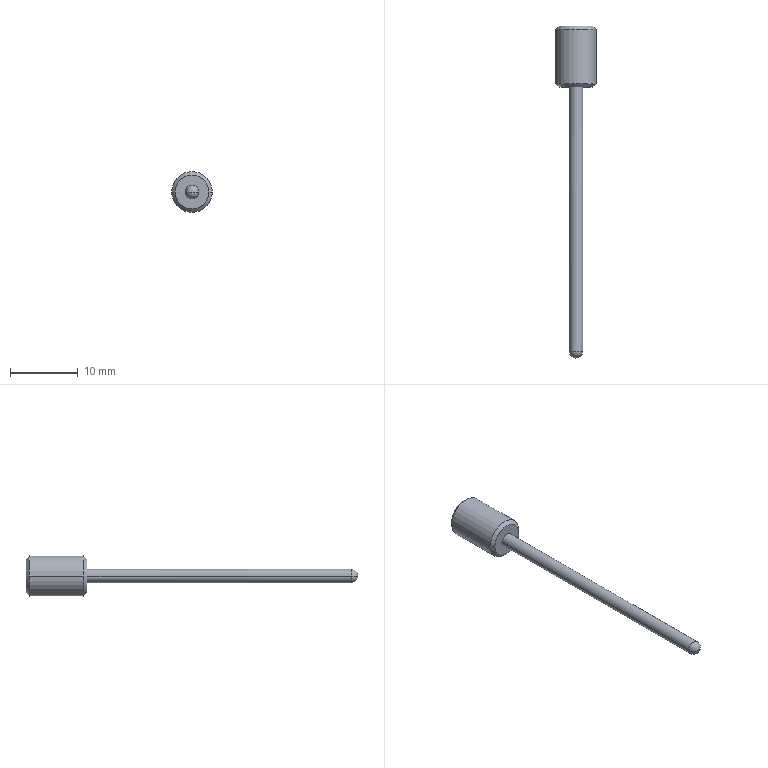Component | SolidWorks | TeaSortingRod-1 | 1 solid | 16 faces | box 6 x 49 x 6 mm | volume 309 mm3 | cone 6 | cylinder 6 | sphere 2 | plane 2 | commonest cylinder face diameters 3.3 x2 2 x2 6 x2
build123d program:
from build123d import *

# Parameters (mm, degrees)
SKETCH1_R             = 3
BOSS_EXTRUDE1_DEPTH   = 9
SKETCH2_R             = 1
BOSS_EXTRUDE2_DEPTH   = 40
M4_TAPPED_HOLE1_D     = 3.3
M4_TAPPED_HOLE1_DEPTH = 7.1
M4_TAPPED_HOLE1_TIP   = 1.65
FILLET1_R             = 1
CHAMFER1_SIZE         = 0.5


with BuildPart() as part:
    # Sketch1 → Boss-Extrude1 (new body)
    with BuildSketch(Plane.XY):
        Circle(SKETCH1_R)
    extrude(amount=BOSS_EXTRUDE1_DEPTH)

    # Sketch2 → Boss-Extrude2 (add)
    with BuildSketch(Plane.XY.offset(9)):
        Circle(SKETCH2_R)
    extrude(amount=BOSS_EXTRUDE2_DEPTH)

    # M4 Tapped Hole1
    with Locations(Plane(origin=(0, 0, 0), x_dir=(-1, 0, 0), z_dir=(0, 0, -1))):
        with Locations((0, 0)):
            Hole(M4_TAPPED_HOLE1_D / 2, depth=M4_TAPPED_HOLE1_DEPTH)
            with Locations((0, 0, -(M4_TAPPED_HOLE1_DEPTH + M4_TAPPED_HOLE1_TIP / 2))):  # 90° drill point
                Cone(0, M4_TAPPED_HOLE1_D / 2, M4_TAPPED_HOLE1_TIP, mode=Mode.SUBTRACT)

    # Fillet1
    fillet1_edges = [part.edges().sort_by_distance(p)[0] for p in [
        (-1, 0, 49),
    ]]
    fillet(fillet1_edges, radius=FILLET1_R)

    # Chamfer1
    chamfer1_edges = [part.edges().sort_by_distance(p)[0] for p in [
        (-3, 0, 0),
        (-3, 0, 9),
    ]]
    chamfer(chamfer1_edges, length=CHAMFER1_SIZE)


solid = part.part

# Placed as in the assembly
solid = solid.moved(Location((64.354, -142.761, 166.933), (90, 0, 0)))
STEP:
#1=COLOUR_RGB('',0.7922,0.8196,0.9333);
#2=FILL_AREA_STYLE_COLOUR('',#1);
#3=FILL_AREA_STYLE('',(#2));
#4=SURFACE_STYLE_FILL_AREA(#3);
#5=SURFACE_SIDE_STYLE('',(#4));
#6=SURFACE_STYLE_USAGE(.BOTH.,#5);
#7=PRESENTATION_STYLE_ASSIGNMENT((#6));
#8=CARTESIAN_POINT('',(2.632,-5.975,6.572));
#9=VERTEX_POINT('',#8);
#10=CARTESIAN_POINT('',(2.435,-5.975,6.572));
#11=VERTEX_POINT('',#10);
#12=CARTESIAN_POINT('',(2.534,-5.975,6.572));
#13=DIRECTION('',(-0.,-1.,-0.));
#14=DIRECTION('',(1.,0.,0.));
#15=AXIS2_PLACEMENT_3D('',#12,#13,#14);
#16=CIRCLE('',#15,0.09843);
#17=EDGE_CURVE('',#9,#11,#16,.T.);
#18=ORIENTED_EDGE('',*,*,#17,.F.);
#19=CARTESIAN_POINT('',(2.652,-5.955,6.572));
#20=VERTEX_POINT('',#19);
#21=CARTESIAN_POINT('',(2.632,-5.975,6.572));
#22=DIRECTION('',(0.7071,0.7071,0.));
#23=VECTOR('',#22,39.37);
#24=LINE('',#21,#23);
#25=EDGE_CURVE('',#9,#20,#24,.T.);
#26=ORIENTED_EDGE('',*,*,#25,.T.);
#27=CARTESIAN_POINT('',(2.416,-5.955,6.572));
#28=VERTEX_POINT('',#27);
#29=CARTESIAN_POINT('',(2.534,-5.955,6.572));
#30=DIRECTION('',(0.,1.,0.));
#31=DIRECTION('',(1.,0.,0.));
#32=AXIS2_PLACEMENT_3D('',#29,#30,#31);
#33=CIRCLE('',#32,0.1181);
#34=EDGE_CURVE('',#28,#20,#33,.T.);
#35=ORIENTED_EDGE('',*,*,#34,.F.);
#36=CARTESIAN_POINT('',(2.435,-5.975,6.572));
#37=DIRECTION('',(-0.7071,0.7071,-0.));
#38=VECTOR('',#37,39.37);
#39=LINE('',#36,#38);
#40=EDGE_CURVE('',#11,#28,#39,.T.);
#41=ORIENTED_EDGE('',*,*,#40,.F.);
#42=EDGE_LOOP('',(#18,#26,#35,#41));
#43=FACE_OUTER_BOUND('',#42,.T.);
#44=CARTESIAN_POINT('',(2.534,-5.975,6.572));
#45=DIRECTION('',(0.,1.,0.));
#46=DIRECTION('',(-1.,0.,0.));
#47=AXIS2_PLACEMENT_3D('',#44,#45,#46);
#48=CONICAL_SURFACE('',#47,0.09843,0.7854);
#49=ADVANCED_FACE('',(#43),#48,.T.);
#50=CARTESIAN_POINT('',(2.435,-5.621,6.572));
#51=VERTEX_POINT('',#50);
#52=CARTESIAN_POINT('',(2.632,-5.621,6.572));
#53=VERTEX_POINT('',#52);
#54=CARTESIAN_POINT('',(2.534,-5.621,6.572));
#55=DIRECTION('',(0.,1.,0.));
#56=DIRECTION('',(1.,0.,0.));
#57=AXIS2_PLACEMENT_3D('',#54,#55,#56);
#58=CIRCLE('',#57,0.09843);
#59=EDGE_CURVE('',#51,#53,#58,.T.);
#60=ORIENTED_EDGE('',*,*,#59,.F.);
#61=CARTESIAN_POINT('',(2.416,-5.64,6.572));
#62=VERTEX_POINT('',#61);
#63=CARTESIAN_POINT('',(2.416,-5.64,6.572));
#64=DIRECTION('',(-0.7071,-0.7071,-0.));
#65=VECTOR('',#64,39.37);
#66=LINE('',#63,#65);
#67=EDGE_CURVE('',#51,#62,#66,.T.);
#68=ORIENTED_EDGE('',*,*,#67,.T.);
#69=CARTESIAN_POINT('',(2.652,-5.64,6.572));
#70=VERTEX_POINT('',#69);
#71=CARTESIAN_POINT('',(2.534,-5.64,6.572));
#72=DIRECTION('',(-0.,-1.,-0.));
#73=DIRECTION('',(1.,0.,0.));
#74=AXIS2_PLACEMENT_3D('',#71,#72,#73);
#75=CIRCLE('',#74,0.1181);
#76=EDGE_CURVE('',#70,#62,#75,.T.);
#77=ORIENTED_EDGE('',*,*,#76,.F.);
#78=CARTESIAN_POINT('',(2.652,-5.64,6.572));
#79=DIRECTION('',(0.7071,-0.7071,0.));
#80=VECTOR('',#79,39.37);
#81=LINE('',#78,#80);
#82=EDGE_CURVE('',#53,#70,#81,.T.);
#83=ORIENTED_EDGE('',*,*,#82,.F.);
#84=EDGE_LOOP('',(#60,#68,#77,#83));
#85=FACE_OUTER_BOUND('',#84,.T.);
#86=CARTESIAN_POINT('',(2.534,-5.64,6.572));
#87=DIRECTION('',(-0.,-1.,-0.));
#88=DIRECTION('',(1.,0.,0.));
#89=AXIS2_PLACEMENT_3D('',#86,#87,#88);
#90=CONICAL_SURFACE('',#89,0.1181,0.7854);
#91=ADVANCED_FACE('',(#85),#90,.T.);
#92=CARTESIAN_POINT('',(2.494,-7.51,6.572));
#93=VERTEX_POINT('',#92);
#94=CARTESIAN_POINT('',(2.573,-7.51,6.572));
#95=VERTEX_POINT('',#94);
#96=CARTESIAN_POINT('',(2.534,-7.51,6.572));
#97=DIRECTION('',(0.,1.,0.));
#98=DIRECTION('',(-1.,0.,0.));
#99=AXIS2_PLACEMENT_3D('',#96,#97,#98);
#100=CIRCLE('',#99,0.03937);
#101=EDGE_CURVE('',#93,#95,#100,.T.);
#102=ORIENTED_EDGE('',*,*,#101,.F.);
#103=CARTESIAN_POINT('',(2.534,-7.55,6.572));
#104=VERTEX_POINT('',#103);
#105=CARTESIAN_POINT('',(2.534,-7.51,6.572));
#106=DIRECTION('',(-0.,-0.,1.));
#107=DIRECTION('',(1.,0.,0.));
#108=AXIS2_PLACEMENT_3D('',#105,#106,#107);
#109=CIRCLE('',#108,0.03937);
#110=EDGE_CURVE('',#93,#104,#109,.T.);
#111=ORIENTED_EDGE('',*,*,#110,.T.);
#112=CARTESIAN_POINT('',(2.534,-7.51,6.572));
#113=DIRECTION('',(0.,0.,-1.));
#114=DIRECTION('',(-1.,0.,0.));
#115=AXIS2_PLACEMENT_3D('',#112,#113,#114);
#116=CIRCLE('',#115,0.03937);
#117=EDGE_CURVE('',#95,#104,#116,.T.);
#118=ORIENTED_EDGE('',*,*,#117,.F.);
#119=EDGE_LOOP('',(#102,#111,#118));
#120=FACE_OUTER_BOUND('',#119,.T.);
#121=CARTESIAN_POINT('',(2.534,-7.51,6.572));
#122=DIRECTION('',(0.,-0.,1.));
#123=DIRECTION('',(1.,0.,0.));
#124=AXIS2_PLACEMENT_3D('',#121,#122,#123);
#125=SPHERICAL_SURFACE('',#124,0.03937);
#126=ADVANCED_FACE('',(#120),#125,.T.);
#127=CARTESIAN_POINT('',(2.599,-5.9,6.572));
#128=VERTEX_POINT('',#127);
#129=CARTESIAN_POINT('',(2.469,-5.9,6.572));
#130=VERTEX_POINT('',#129);
#131=CARTESIAN_POINT('',(2.534,-5.9,6.572));
#132=DIRECTION('',(0.,1.,0.));
#133=DIRECTION('',(-1.,0.,0.));
#134=AXIS2_PLACEMENT_3D('',#131,#132,#133);
#135=CIRCLE('',#134,0.06496);
#136=EDGE_CURVE('',#128,#130,#135,.T.);
#137=ORIENTED_EDGE('',*,*,#136,.F.);
#138=CARTESIAN_POINT('',(2.599,-5.621,6.572));
#139=VERTEX_POINT('',#138);
#140=CARTESIAN_POINT('',(2.599,-5.621,6.572));
#141=DIRECTION('',(0.,1.,0.));
#142=VECTOR('',#141,39.37);
#143=LINE('',#140,#142);
#144=EDGE_CURVE('',#128,#139,#143,.T.);
#145=ORIENTED_EDGE('',*,*,#144,.T.);
#146=CARTESIAN_POINT('',(2.469,-5.621,6.572));
#147=VERTEX_POINT('',#146);
#148=CARTESIAN_POINT('',(2.534,-5.621,6.572));
#149=DIRECTION('',(0.,1.,0.));
#150=DIRECTION('',(-1.,0.,0.));
#151=AXIS2_PLACEMENT_3D('',#148,#149,#150);
#152=CIRCLE('',#151,0.06496);
#153=EDGE_CURVE('',#139,#147,#152,.T.);
#154=ORIENTED_EDGE('',*,*,#153,.T.);
#155=CARTESIAN_POINT('',(2.469,-5.621,6.572));
#156=DIRECTION('',(0.,1.,0.));
#157=VECTOR('',#156,39.37);
#158=LINE('',#155,#157);
#159=EDGE_CURVE('',#130,#147,#158,.T.);
#160=ORIENTED_EDGE('',*,*,#159,.F.);
#161=EDGE_LOOP('',(#137,#145,#154,#160));
#162=FACE_OUTER_BOUND('',#161,.T.);
#163=CARTESIAN_POINT('',(2.534,-5.621,6.572));
#164=DIRECTION('',(0.,1.,0.));
#165=DIRECTION('',(-1.,0.,0.));
#166=AXIS2_PLACEMENT_3D('',#163,#164,#165);
#167=CYLINDRICAL_SURFACE('',#166,0.06496);
#168=ADVANCED_FACE('',(#162),#167,.F.);
#169=CARTESIAN_POINT('',(2.534,-5.965,6.572));
#170=VERTEX_POINT('',#169);
#171=CARTESIAN_POINT('',(2.469,-5.9,6.572));
#172=DIRECTION('',(-0.7071,0.7071,-0.));
#173=VECTOR('',#172,39.37);
#174=LINE('',#171,#173);
#175=EDGE_CURVE('',#170,#130,#174,.T.);
#176=ORIENTED_EDGE('',*,*,#175,.F.);
#177=CARTESIAN_POINT('',(2.599,-5.9,6.572));
#178=DIRECTION('',(0.7071,0.7071,0.));
#179=VECTOR('',#178,39.37);
#180=LINE('',#177,#179);
#181=EDGE_CURVE('',#170,#128,#180,.T.);
#182=ORIENTED_EDGE('',*,*,#181,.T.);
#183=ORIENTED_EDGE('',*,*,#136,.T.);
#184=EDGE_LOOP('',(#176,#182,#183));
#185=FACE_OUTER_BOUND('',#184,.T.);
#186=CARTESIAN_POINT('',(2.534,-5.9,6.572));
#187=DIRECTION('',(0.,1.,0.));
#188=DIRECTION('',(-1.,0.,0.));
#189=AXIS2_PLACEMENT_3D('',#186,#187,#188);
#190=CONICAL_SURFACE('',#189,0.06496,0.7854);
#191=ADVANCED_FACE('',(#185),#190,.F.);
#192=ORIENTED_EDGE('',*,*,#101,.T.);
#193=CARTESIAN_POINT('',(2.573,-5.975,6.572));
#194=VERTEX_POINT('',#193);
#195=CARTESIAN_POINT('',(2.573,-7.55,6.572));
#196=DIRECTION('',(0.,1.,0.));
#197=VECTOR('',#196,39.37);
#198=LINE('',#195,#197);
#199=EDGE_CURVE('',#95,#194,#198,.T.);
#200=ORIENTED_EDGE('',*,*,#199,.T.);
#201=CARTESIAN_POINT('',(2.494,-5.975,6.572));
#202=VERTEX_POINT('',#201);
#203=CARTESIAN_POINT('',(2.534,-5.975,6.572));
#204=DIRECTION('',(-0.,-1.,-0.));
#205=DIRECTION('',(1.,0.,0.));
#206=AXIS2_PLACEMENT_3D('',#203,#204,#205);
#207=CIRCLE('',#206,0.03937);
#208=EDGE_CURVE('',#194,#202,#207,.T.);
#209=ORIENTED_EDGE('',*,*,#208,.T.);
#210=CARTESIAN_POINT('',(2.494,-7.55,6.572));
#211=DIRECTION('',(0.,1.,0.));
#212=VECTOR('',#211,39.37);
#213=LINE('',#210,#212);
#214=EDGE_CURVE('',#93,#202,#213,.T.);
#215=ORIENTED_EDGE('',*,*,#214,.F.);
#216=EDGE_LOOP('',(#192,#200,#209,#215));
#217=FACE_OUTER_BOUND('',#216,.T.);
#218=CARTESIAN_POINT('',(2.534,-7.55,6.572));
#219=DIRECTION('',(0.,1.,0.));
#220=DIRECTION('',(-1.,0.,0.));
#221=AXIS2_PLACEMENT_3D('',#218,#219,#220);
#222=CYLINDRICAL_SURFACE('',#221,0.03937);
#223=ADVANCED_FACE('',(#217),#222,.T.);
#224=ORIENTED_EDGE('',*,*,#34,.T.);
#225=CARTESIAN_POINT('',(2.652,-5.975,6.572));
#226=DIRECTION('',(0.,1.,0.));
#227=VECTOR('',#226,39.37);
#228=LINE('',#225,#227);
#229=EDGE_CURVE('',#20,#70,#228,.T.);
#230=ORIENTED_EDGE('',*,*,#229,.T.);
#231=ORIENTED_EDGE('',*,*,#76,.T.);
#232=CARTESIAN_POINT('',(2.416,-5.975,6.572));
#233=DIRECTION('',(0.,1.,0.));
#234=VECTOR('',#233,39.37);
#235=LINE('',#232,#234);
#236=EDGE_CURVE('',#28,#62,#235,.T.);
#237=ORIENTED_EDGE('',*,*,#236,.F.);
#238=EDGE_LOOP('',(#224,#230,#231,#237));
#239=FACE_OUTER_BOUND('',#238,.T.);
#240=CARTESIAN_POINT('',(2.534,-5.975,6.572));
#241=DIRECTION('',(0.,1.,0.));
#242=DIRECTION('',(-1.,0.,0.));
#243=AXIS2_PLACEMENT_3D('',#240,#241,#242);
#244=CYLINDRICAL_SURFACE('',#243,0.1181);
#245=ADVANCED_FACE('',(#239),#244,.T.);
#246=CARTESIAN_POINT('',(2.534,-5.975,6.572));
#247=DIRECTION('',(-0.,-1.,-0.));
#248=DIRECTION('',(1.,0.,0.));
#249=AXIS2_PLACEMENT_3D('',#246,#247,#248);
#250=CIRCLE('',#249,0.09843);
#251=EDGE_CURVE('',#11,#9,#250,.T.);
#252=ORIENTED_EDGE('',*,*,#251,.T.);
#253=ORIENTED_EDGE('',*,*,#17,.T.);
#254=EDGE_LOOP('',(#252,#253));
#255=FACE_OUTER_BOUND('',#254,.T.);
#256=CARTESIAN_POINT('',(2.534,-5.975,6.572));
#257=DIRECTION('',(-0.,-1.,-0.));
#258=DIRECTION('',(1.,0.,0.));
#259=AXIS2_PLACEMENT_3D('',#256,#257,#258);
#260=CIRCLE('',#259,0.03937);
#261=EDGE_CURVE('',#202,#194,#260,.T.);
#262=ORIENTED_EDGE('',*,*,#261,.F.);
#263=ORIENTED_EDGE('',*,*,#208,.F.);
#264=EDGE_LOOP('',(#262,#263));
#265=FACE_BOUND('',#264,.T.);
#266=CARTESIAN_POINT('',(2.534,-5.975,6.572));
#267=DIRECTION('',(-0.,-1.,-0.));
#268=DIRECTION('',(1.,-0.,0.));
#269=AXIS2_PLACEMENT_3D('',#266,#267,#268);
#270=PLANE('',#269);
#271=ADVANCED_FACE('',(#255,#265),#270,.T.);
#272=ORIENTED_EDGE('',*,*,#229,.F.);
#273=CARTESIAN_POINT('',(2.534,-5.955,6.572));
#274=DIRECTION('',(0.,1.,0.));
#275=DIRECTION('',(1.,0.,0.));
#276=AXIS2_PLACEMENT_3D('',#273,#274,#275);
#277=CIRCLE('',#276,0.1181);
#278=EDGE_CURVE('',#20,#28,#277,.T.);
#279=ORIENTED_EDGE('',*,*,#278,.T.);
#280=ORIENTED_EDGE('',*,*,#236,.T.);
#281=CARTESIAN_POINT('',(2.534,-5.64,6.572));
#282=DIRECTION('',(-0.,-1.,-0.));
#283=DIRECTION('',(1.,0.,0.));
#284=AXIS2_PLACEMENT_3D('',#281,#282,#283);
#285=CIRCLE('',#284,0.1181);
#286=EDGE_CURVE('',#62,#70,#285,.T.);
#287=ORIENTED_EDGE('',*,*,#286,.T.);
#288=EDGE_LOOP('',(#272,#279,#280,#287));
#289=FACE_OUTER_BOUND('',#288,.T.);
#290=CARTESIAN_POINT('',(2.534,-5.975,6.572));
#291=DIRECTION('',(0.,1.,0.));
#292=DIRECTION('',(-1.,0.,0.));
#293=AXIS2_PLACEMENT_3D('',#290,#291,#292);
#294=CYLINDRICAL_SURFACE('',#293,0.1181);
#295=ADVANCED_FACE('',(#289),#294,.T.);
#296=CARTESIAN_POINT('',(2.534,-5.621,6.572));
#297=DIRECTION('',(0.,1.,0.));
#298=DIRECTION('',(1.,0.,0.));
#299=AXIS2_PLACEMENT_3D('',#296,#297,#298);
#300=CIRCLE('',#299,0.09843);
#301=EDGE_CURVE('',#53,#51,#300,.T.);
#302=ORIENTED_EDGE('',*,*,#301,.T.);
#303=ORIENTED_EDGE('',*,*,#59,.T.);
#304=EDGE_LOOP('',(#302,#303));
#305=FACE_OUTER_BOUND('',#304,.T.);
#306=CARTESIAN_POINT('',(2.534,-5.621,6.572));
#307=DIRECTION('',(0.,1.,0.));
#308=DIRECTION('',(-1.,0.,0.));
#309=AXIS2_PLACEMENT_3D('',#306,#307,#308);
#310=CIRCLE('',#309,0.06496);
#311=EDGE_CURVE('',#147,#139,#310,.T.);
#312=ORIENTED_EDGE('',*,*,#311,.F.);
#313=ORIENTED_EDGE('',*,*,#153,.F.);
#314=EDGE_LOOP('',(#312,#313));
#315=FACE_BOUND('',#314,.T.);
#316=CARTESIAN_POINT('',(2.534,-5.621,6.572));
#317=DIRECTION('',(-0.,-1.,-0.));
#318=DIRECTION('',(1.,-0.,0.));
#319=AXIS2_PLACEMENT_3D('',#316,#317,#318);
#320=PLANE('',#319);
#321=ADVANCED_FACE('',(#305,#315),#320,.F.);
#322=ORIENTED_EDGE('',*,*,#199,.F.);
#323=CARTESIAN_POINT('',(2.534,-7.51,6.572));
#324=DIRECTION('',(0.,1.,0.));
#325=DIRECTION('',(-1.,0.,0.));
#326=AXIS2_PLACEMENT_3D('',#323,#324,#325);
#327=CIRCLE('',#326,0.03937);
#328=EDGE_CURVE('',#95,#93,#327,.T.);
#329=ORIENTED_EDGE('',*,*,#328,.T.);
#330=ORIENTED_EDGE('',*,*,#214,.T.);
#331=ORIENTED_EDGE('',*,*,#261,.T.);
#332=EDGE_LOOP('',(#322,#329,#330,#331));
#333=FACE_OUTER_BOUND('',#332,.T.);
#334=CARTESIAN_POINT('',(2.534,-7.55,6.572));
#335=DIRECTION('',(0.,1.,0.));
#336=DIRECTION('',(-1.,0.,0.));
#337=AXIS2_PLACEMENT_3D('',#334,#335,#336);
#338=CYLINDRICAL_SURFACE('',#337,0.03937);
#339=ADVANCED_FACE('',(#333),#338,.T.);
#340=ORIENTED_EDGE('',*,*,#181,.F.);
#341=ORIENTED_EDGE('',*,*,#175,.T.);
#342=CARTESIAN_POINT('',(2.534,-5.9,6.572));
#343=DIRECTION('',(0.,1.,0.));
#344=DIRECTION('',(-1.,0.,0.));
#345=AXIS2_PLACEMENT_3D('',#342,#343,#344);
#346=CIRCLE('',#345,0.06496);
#347=EDGE_CURVE('',#130,#128,#346,.T.);
#348=ORIENTED_EDGE('',*,*,#347,.T.);
#349=EDGE_LOOP('',(#340,#341,#348));
#350=FACE_OUTER_BOUND('',#349,.T.);
#351=CARTESIAN_POINT('',(2.534,-5.9,6.572));
#352=DIRECTION('',(0.,1.,0.));
#353=DIRECTION('',(-1.,0.,0.));
#354=AXIS2_PLACEMENT_3D('',#351,#352,#353);
#355=CONICAL_SURFACE('',#354,0.06496,0.7854);
#356=ADVANCED_FACE('',(#350),#355,.F.);
#357=ORIENTED_EDGE('',*,*,#144,.F.);
#358=ORIENTED_EDGE('',*,*,#347,.F.);
#359=ORIENTED_EDGE('',*,*,#159,.T.);
#360=ORIENTED_EDGE('',*,*,#311,.T.);
#361=EDGE_LOOP('',(#357,#358,#359,#360));
#362=FACE_OUTER_BOUND('',#361,.T.);
#363=CARTESIAN_POINT('',(2.534,-5.621,6.572));
#364=DIRECTION('',(0.,1.,0.));
#365=DIRECTION('',(-1.,0.,0.));
#366=AXIS2_PLACEMENT_3D('',#363,#364,#365);
#367=CYLINDRICAL_SURFACE('',#366,0.06496);
#368=ADVANCED_FACE('',(#362),#367,.F.);
#369=ORIENTED_EDGE('',*,*,#110,.F.);
#370=ORIENTED_EDGE('',*,*,#328,.F.);
#371=ORIENTED_EDGE('',*,*,#117,.T.);
#372=EDGE_LOOP('',(#369,#370,#371));
#373=FACE_OUTER_BOUND('',#372,.T.);
#374=CARTESIAN_POINT('',(2.534,-7.51,6.572));
#375=DIRECTION('',(0.,-0.,1.));
#376=DIRECTION('',(1.,0.,0.));
#377=AXIS2_PLACEMENT_3D('',#374,#375,#376);
#378=SPHERICAL_SURFACE('',#377,0.03937);
#379=ADVANCED_FACE('',(#373),#378,.T.);
#380=ORIENTED_EDGE('',*,*,#67,.F.);
#381=ORIENTED_EDGE('',*,*,#301,.F.);
#382=ORIENTED_EDGE('',*,*,#82,.T.);
#383=ORIENTED_EDGE('',*,*,#286,.F.);
#384=EDGE_LOOP('',(#380,#381,#382,#383));
#385=FACE_OUTER_BOUND('',#384,.T.);
#386=CARTESIAN_POINT('',(2.534,-5.64,6.572));
#387=DIRECTION('',(-0.,-1.,-0.));
#388=DIRECTION('',(1.,0.,0.));
#389=AXIS2_PLACEMENT_3D('',#386,#387,#388);
#390=CONICAL_SURFACE('',#389,0.1181,0.7854);
#391=ADVANCED_FACE('',(#385),#390,.T.);
#392=ORIENTED_EDGE('',*,*,#25,.F.);
#393=ORIENTED_EDGE('',*,*,#251,.F.);
#394=ORIENTED_EDGE('',*,*,#40,.T.);
#395=ORIENTED_EDGE('',*,*,#278,.F.);
#396=EDGE_LOOP('',(#392,#393,#394,#395));
#397=FACE_OUTER_BOUND('',#396,.T.);
#398=CARTESIAN_POINT('',(2.534,-5.975,6.572));
#399=DIRECTION('',(0.,1.,0.));
#400=DIRECTION('',(-1.,0.,0.));
#401=AXIS2_PLACEMENT_3D('',#398,#399,#400);
#402=CONICAL_SURFACE('',#401,0.09843,0.7854);
#403=ADVANCED_FACE('',(#397),#402,.T.);
#404=CLOSED_SHELL('',(#49,#91,#126,#168,#191,#223,#245,#271,#295,#321,#339,#356,#368,#379,#391,#403));
#405=MANIFOLD_SOLID_BREP('',#404);
#406=STYLED_ITEM('',(#7),#405);
#407=(LENGTH_UNIT()NAMED_UNIT(*)SI_UNIT($,.METRE.));
#408=LENGTH_MEASURE_WITH_UNIT(LENGTH_MEASURE(0.0254),#407);
#409=DIMENSIONAL_EXPONENTS(1.,0.,0.,0.,0.,0.,0.);
#410=(CONVERSION_BASED_UNIT('',#408)LENGTH_UNIT()NAMED_UNIT(#409));
#411=UNCERTAINTY_MEASURE_WITH_UNIT(LENGTH_MEASURE(0.00001),#410,'','');
#412=(NAMED_UNIT(*)PLANE_ANGLE_UNIT()SI_UNIT($,.RADIAN.));
#413=(NAMED_UNIT(*)SI_UNIT($,.STERADIAN.)SOLID_ANGLE_UNIT());
#414=(GEOMETRIC_REPRESENTATION_CONTEXT(3)GLOBAL_UNCERTAINTY_ASSIGNED_CONTEXT((#411))GLOBAL_UNIT_ASSIGNED_CONTEXT((#410,#412,#413))REPRESENTATION_CONTEXT('',''));
#415=MECHANICAL_DESIGN_GEOMETRIC_PRESENTATION_REPRESENTATION('',(#406),#414);
#416=PRESENTATION_LAYER_ASSIGNMENT('','',(#406));
#417=CARTESIAN_POINT('',(0.,0.,0.));
#418=DIRECTION('',(0.,0.,1.));
#419=DIRECTION('',(1.,0.,0.));
#420=AXIS2_PLACEMENT_3D('',#417,#418,#419);
#421=(LENGTH_UNIT()NAMED_UNIT(*)SI_UNIT($,.METRE.));
#422=LENGTH_MEASURE_WITH_UNIT(LENGTH_MEASURE(0.0254),#421);
#423=DIMENSIONAL_EXPONENTS(1.,0.,0.,0.,0.,0.,0.);
#424=(CONVERSION_BASED_UNIT('',#422)LENGTH_UNIT()NAMED_UNIT(#423));
#425=UNCERTAINTY_MEASURE_WITH_UNIT(LENGTH_MEASURE(0.00001),#424,'','');
#426=(NAMED_UNIT(*)PLANE_ANGLE_UNIT()SI_UNIT($,.RADIAN.));
#427=(NAMED_UNIT(*)SI_UNIT($,.STERADIAN.)SOLID_ANGLE_UNIT());
#428=(GEOMETRIC_REPRESENTATION_CONTEXT(3)GLOBAL_UNCERTAINTY_ASSIGNED_CONTEXT((#425))GLOBAL_UNIT_ASSIGNED_CONTEXT((#424,#426,#427))REPRESENTATION_CONTEXT('',''));
#429=ADVANCED_BREP_SHAPE_REPRESENTATION('',(#405,#420),#428);